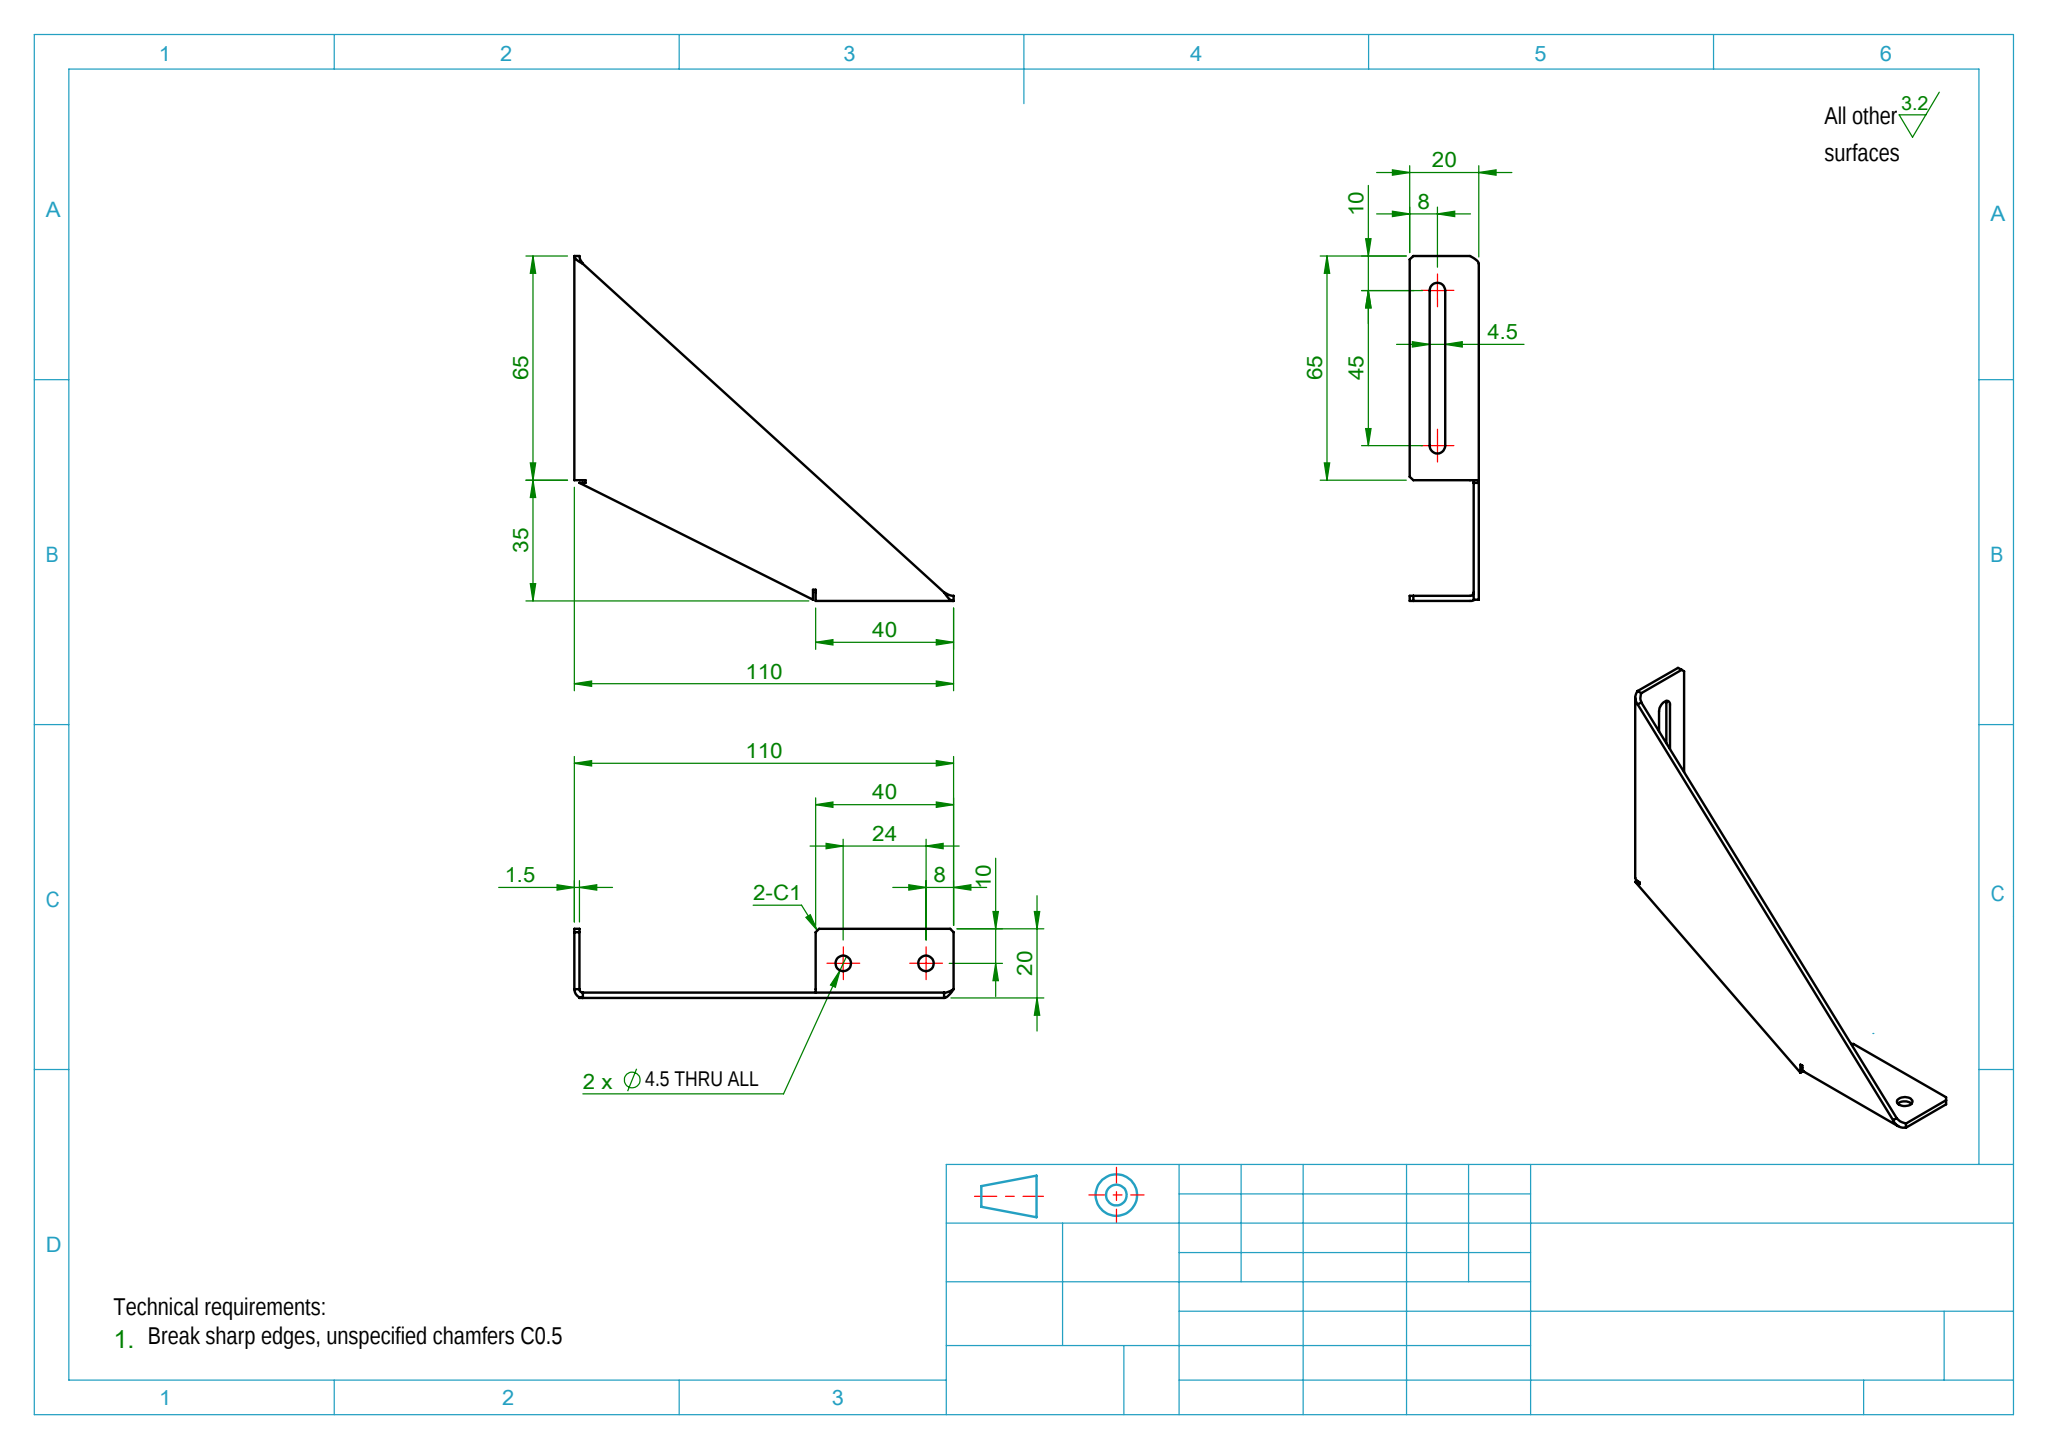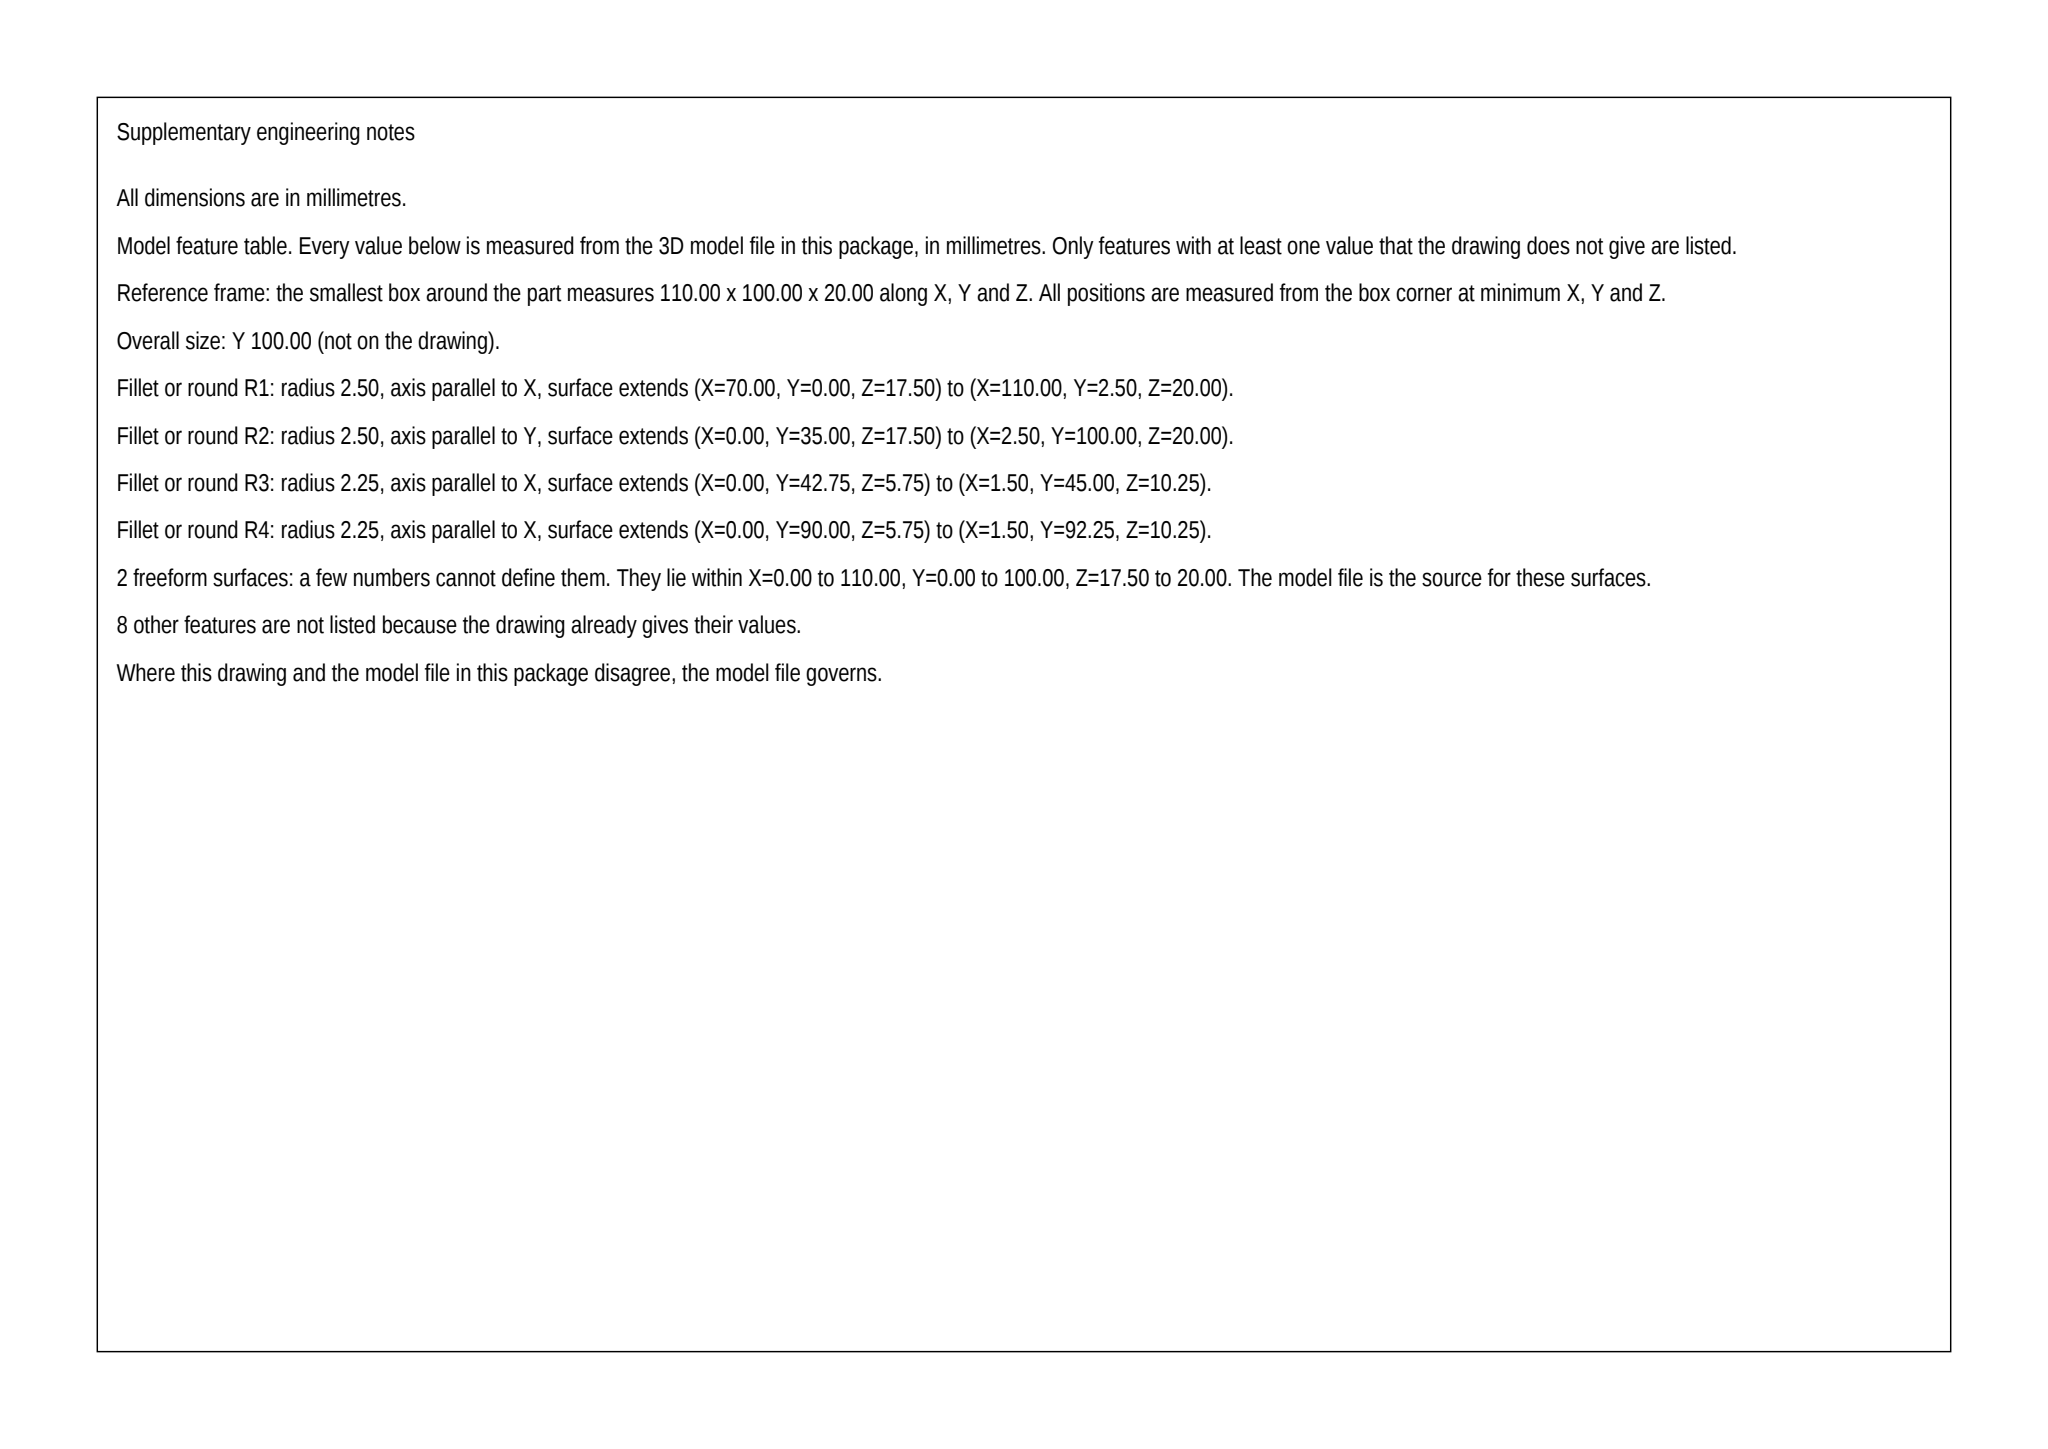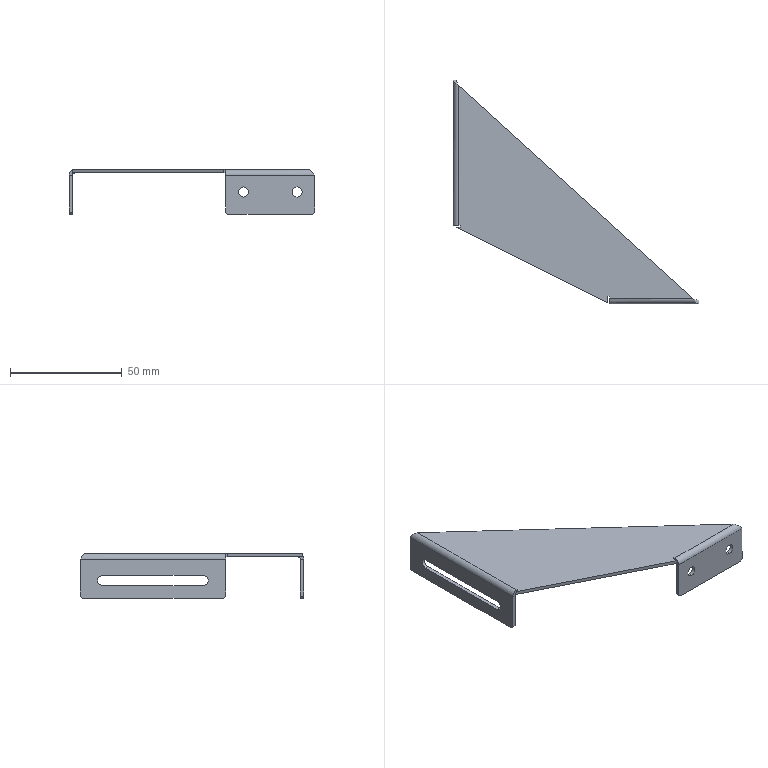Part | SolidWorks | mm | 1 solid | 40 faces | box 110 x 100 x 20 mm | volume 8822 mm3 | plane 28 | cylinder 10 | spline 2 | commonest cylinder face diameters 4.5 x6 5 x2 2 x2
Drawing notes:
ALL 90° BENDS: INNER R1, OUTER R2.5 (MATL T1.5) | from the solid: Cylinders Ø2.0 (axis x @ y2.52,z17.5 L40; axis y @ x2.52,z17.5 L65) = inner R1; Ø5.0 on same axes = outer R2.5; wall planes at 0.02/1.52 give T1.5